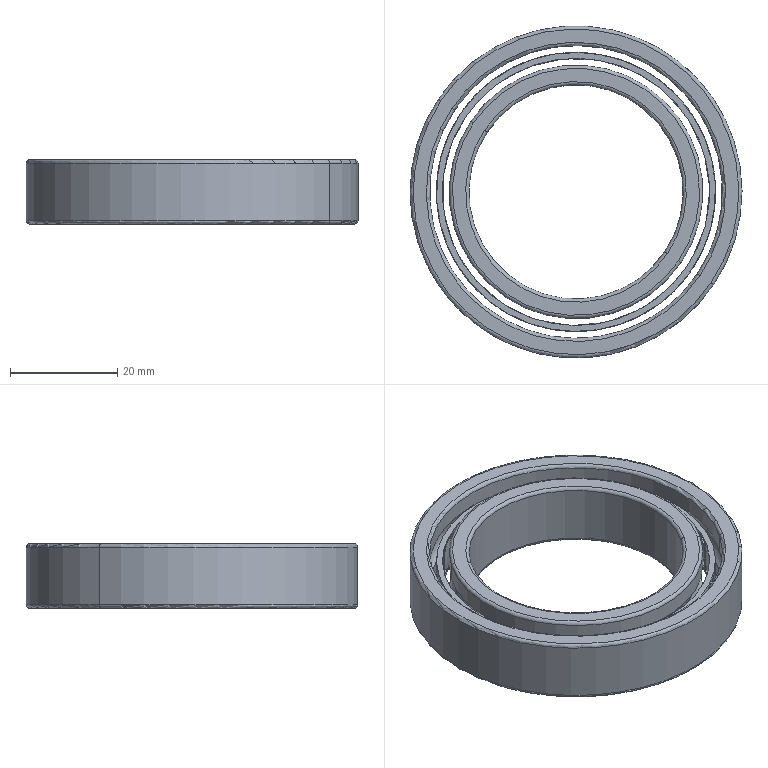Component | SolidWorks | DriveDevice-1_Gb_t276-2013[DeepGrooveBallBearing[60000]61908]-1 | 26 solids | 278 faces | volume 13745 mm3 | cylinder 112 | sphere 92 | plane 52 | torus 22 | commonest cylinder face diameters 6.15 x48 49.9 x26 52.1 x26 47.333 x4 54.667 x4 40 x2 62 x2